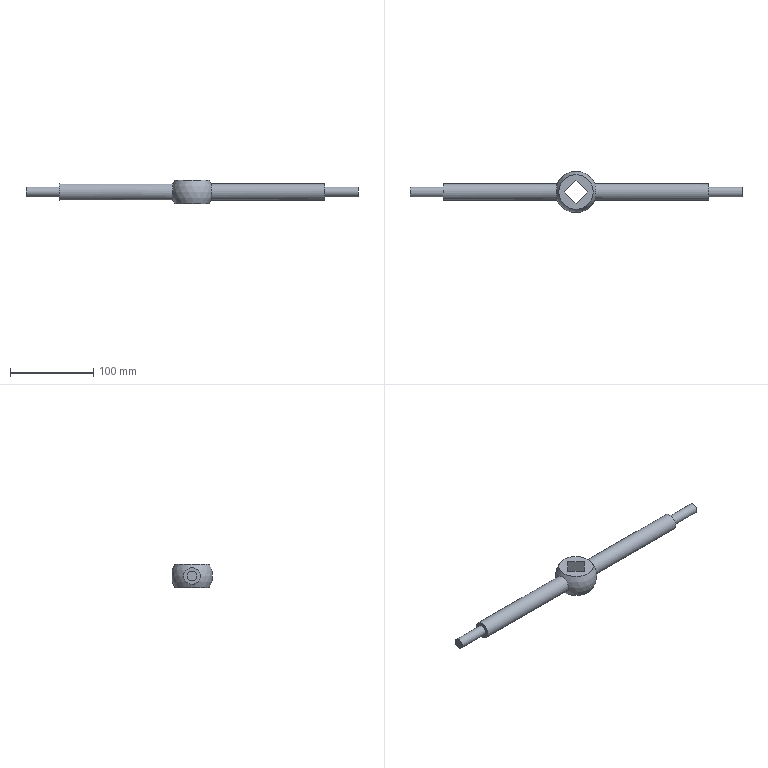Component | NX | GRIP | 1 solid | 15 faces | volume 132548 mm3 | plane 10 | cylinder 4 | sphere 1 | commonest cylinder face diameters 20 x2 12 x2